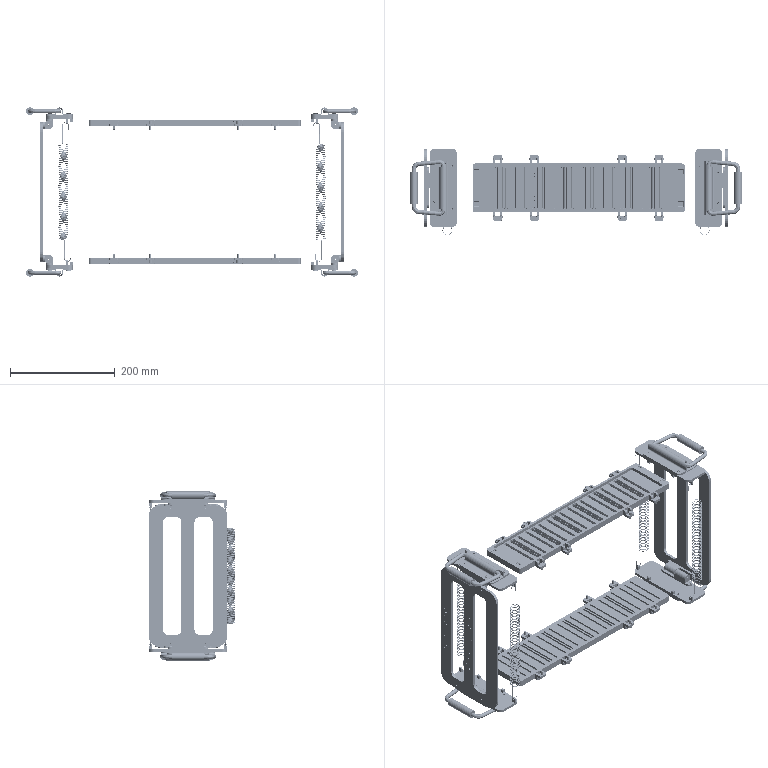Assembly | SolidWorks | mm | 128 component files | 156 solids | 4924 faces | box 634 x 165.5 x 323 mm | volume 1114306 mm3 | plane 2454 | cylinder 1068 | spline 750 | cone 404 | torus 248 | commonest cylinder face diameters 3 x192 3.5 x128 3.4 x96 5.5 x96 5 x72 8 x48 6 x40 2 x40
Bill of materials:
MGL-PACK-01-01WeldPlate1 | 1 |  | Long, thin rectangular plate with rounded corners. The top face has a shallow recessed pocket with many parallel through-slots across the plate's width, plus small square features near the four corners.
MGL-PACK-01-02LocatingBlock | 8 |  | Block with a U-shaped (clevis-like) profile: two upright lugs on a base, each lug with a cross hole. A cylindrical pin with a rounded or chamfered tip sticks out from the underside, and one end of the base is rounded.
MGL-PACK-01-03FixingBlock | 8 |  | U-shaped block similar to the pin-carrying variant: two upright lugs with aligned cross holes, a rounded base end, and a vertical through-hole in the base instead of a protruding pin.
SocketHeadCapScrew_M3_12[GB_T70.1-2000] | 32 |  | Socket-head cap-screw-shaped part: a cylindrical head with a hexagonal socket and a long, plain cylindrical shank with a chamfered tip.
SocketHeadCapScrew_M4_12[GB_T70.1-2000] | 8 |  | Socket-head cap-screw-shaped part with a cylindrical head, a hexagonal socket and a short, plain cylindrical shank with a chamfered end.
MGL-PACK-02-01WeldedPlate2 | 1 |  | Long, thin rectangular plate with rounded corners and many parallel slots spread over its full width, with pairs of small holes on the long edge.
MGL-PACK-03-01FixedPlate | 2 |  | Thin flat frame plate with rounded corners, two large, round-cornered rectangular openings separated by a central bar, and four small holes near the corners.
MGL-PACK-03-02MovingPlate | 4 |  | Flat rectangular plate with fully rounded corners and an asymmetric pattern of round holes: four larger holes, two of them with a smaller hole next to each.
MGL-PACK-03-03SpringSeat | 8 |  | Lug or tab block: rectangular body with a semicircular top end and one large round through-hole centered on the arc.
MGL-PACK-03-04LimitBlock | 8 |  | Solid extruded block with a rectangular lower section and a semicircular or arched top. It has no holes.
MGL-PACK-03-05TensionSpring | 4 |  | Helical coil spring with closely spaced coils and an extended hook formed at each end, consistent with an extension spring.
MGL-PACK-03-06Handle | 4 |  | Folding or drop-style handle: a flat mounting plate with four holes and a curled hinge edge, holding a bent rod in a rectangular U-loop with a cylindrical grip sleeve on the far bar.
MGL-PACK-03-07-01HingePart1 | 4 |  | Flat, thin obround (slot-shaped) plate with a small through-hole near each rounded end. A raised block with a rounded edge (knuckle-like boss) sits on one face along part of the plate's length, offset to one long edge. A slender cylinder (pin) sticks out of the boss end and runs parallel to the plate's long axis, past the boss, for about half the plate length. The overall layout looks like a hinge leaf with a pin.
MGL-PACK-03-07-02HingePart2 | 4 |  | Flat obround plate with a small through-hole near each rounded end. Under one face it has a boss with a rounded end, running along about a third of the plate's length, offset toward one end, with a round through-bore parallel to the plate's long axis. The overall layout looks like a hinge leaf with a knuckle.
PhillipsCountersunkScrewM3_6[GB_T819.1-2000] | 16 |  | Flat-topped countersunk (conical) head with a cross-shaped recess. Below the head is a short necked or filleted transition, then a plain cylindrical shank that ends in a chamfer. The shape looks like a short countersunk screw, but no thread is modeled.
PhillipsCountersunkScrewM5_8[GB_T819.1-2000] | 16 |  | Flat-topped countersunk (conical) head with a cross-shaped recess. Below the head is a necked or filleted transition, then a short plain cylindrical shank that ends in a chamfer. Compared with its head diameter, the shank looks shorter than in unnamed part. The shape looks like a short countersunk screw, but no thread is modeled.
Mates:
1. coincident | MGL-PACK-01-00WeldedPlate1Assembly-1/MGL-PACK-01-01WeldPlate1-1 face at (202.5, 46.5, 12) dir (1, 0, 0) | MGL-PACK-02-00WeldedPlate2Assembly-1/MGL-PACK-02-01WeldedPlate2-1 face at (202.5, 46.5, -263.6) dir (1, 0, 0)
2. coincident | MGL-PACK-01-00WeldedPlate1Assembly-1/MGL-PACK-01-01WeldPlate1-1 face at (-202.5, 46.5, 12) dir (0, 1, 0) | MGL-PACK-02-00WeldedPlate2Assembly-1/MGL-PACK-02-01WeldedPlate2-1 face at (202.5, 46.5, -263.6) dir (0, 1, 0)
3. distance | MGL-PACK-02-00WeldedPlate2Assembly-1/MGL-PACK-02-01WeldedPlate2-1 face at (0, 0, -251.6) dir (0, 0, 1) | MGL-PACK-01-00WeldedPlate1Assembly-1/MGL-PACK-01-01WeldPlate1-1 face at (0, 0, 0) dir (0, 0, -1)
4. distance | MGL-PACK-01-00WeldedPlate1Assembly-1/MGL-PACK-01-01WeldPlate1-1 face at (-202.5, 46.5, 12) dir (0, 1, 0) | MGL-PACK-03-00Fixture-1/MGL-PACK-03-02MovingPlate-1 face at (222.5, 75, 13.7) dir (0, 1, 0)
5. distance | MGL-PACK-03-00Fixture-1/MGL-PACK-03-02MovingPlate-2 face at (222.5, 75, -265.3) dir (-1, 0, 0) | MGL-PACK-02-00WeldedPlate2Assembly-1/MGL-PACK-02-01WeldedPlate2-1 face at (202.5, 46.5, -263.6) dir (1, 0, 0)
6. distance | MGL-PACK-03-00Fixture-2/MGL-PACK-03-02MovingPlate-2 face at (-232.5, 75, 13.7) dir (1, 0, 0) | MGL-PACK-01-00WeldedPlate1Assembly-1/MGL-PACK-01-01WeldPlate1-1 face at (-202.5, 46.5, 12) dir (-1, 0, 0)
7. distance | MGL-PACK-01-00WeldedPlate1Assembly-1/MGL-PACK-01-01WeldPlate1-1 face at (0, 0, 12) dir (0, 0, 1) | MGL-PACK-03-00Fixture-2/MGL-PACK-03-02MovingPlate-2 face at (-258.5, 0, 13.7) dir (0, 0, -1)
8. distance | MGL-PACK-03-00Fixture-1/MGL-PACK-03-02MovingPlate-2 face at (248.5, 0, -265.3) dir (0, 0, 1) | MGL-PACK-02-00WeldedPlate2Assembly-1/MGL-PACK-02-01WeldedPlate2-1 face at (0, 0, -263.6) dir (0, 0, -1)
9. distance | MGL-PACK-01-00WeldedPlate1Assembly-1/MGL-PACK-01-01WeldPlate1-1 face at (-202.5, 46.5, 12) dir (0, 1, 0) | MGL-PACK-03-00Fixture-2/MGL-PACK-03-01FixedPlate-1 face at (-289.5, 75, 8.7) dir (0, 1, 0)
10. coincident | MGL-PACK-01-01WeldPlate1-1 face at (-202.5, 46.5, 12) dir (0, 1, 0) | MGL-PACK-01-02LocatingBlock-1 face at (-163.05, 46.5, 12) dir (0, -1, 0)
11. concentric | MGL-PACK-01-01WeldPlate1-1 face at (-161.05, 46.5, 8.5) dir (0, 1, 0) r 1.5 | MGL-PACK-01-02LocatingBlock-1 face at (-161.05, 53.5, 8.5) dir (0, 1, 0) r 1.7
12. concentric | MGL-PACK-01-01WeldPlate1-1 face at (-148.05, 46.5, 8.5) dir (0, 1, 0) r 1.5 | MGL-PACK-01-02LocatingBlock-1 face at (-148.05, 53.5, 8.5) dir (0, 1, 0) r 1.7
13. coincident | MGL-PACK-01-01WeldPlate1-1 face at (-202.5, 46.5, 12) dir (0, 1, 0) | MGL-PACK-01-02LocatingBlock-9 face at (157.95, 46.5, 12) dir (0, -1, 0)
14. concentric | MGL-PACK-01-01WeldPlate1-1 face at (146.95, 46.5, 8.5) dir (0, 1, 0) r 1.5 | MGL-PACK-01-02LocatingBlock-9 face at (146.95, 53.5, 8.5) dir (0, 1, 0) r 1.7
15. concentric | MGL-PACK-01-01WeldPlate1-1 face at (159.95, 46.5, 8.5) dir (0, 1, 0) r 1.5 | MGL-PACK-01-02LocatingBlock-9 face at (159.95, 53.5, 8.5) dir (0, 1, 0) r 1.7
16. coincident | MGL-PACK-01-01WeldPlate1-1 face at (-202.5, 46.5, 12) dir (0, 1, 0) | MGL-PACK-01-03FixingBlock-1 face at (-93.05, 46.5, 12) dir (0, -1, 0)
17. coincident | MGL-PACK-01-01WeldPlate1-1 face at (-202.5, 46.5, 12) dir (0, 1, 0) | MGL-PACK-01-03FixingBlock-2 face at (87.95, 46.5, 12) dir (0, -1, 0)
18. coincident | MGL-PACK-01-01WeldPlate1-1 face at (-202.5, -46.5, 12) dir (0, -1, 0) | MGL-PACK-01-03FixingBlock-3 face at (-89.05, -46.5, 12) dir (0, 1, 0)
19. coincident | MGL-PACK-01-01WeldPlate1-1 face at (-202.5, -46.5, 12) dir (0, -1, 0) | MGL-PACK-01-03FixingBlock-4 face at (78.95, -46.5, 12) dir (0, 1, 0)
20. concentric | MGL-PACK-01-01WeldPlate1-1 face at (-91.05, 46.5, 8.5) dir (0, 1, 0) r 1.5 | MGL-PACK-01-03FixingBlock-1 face at (-91.05, 53.5, 8.5) dir (0, 1, 0) r 1.7
21. concentric | MGL-PACK-01-01WeldPlate1-1 face at (-78.05, 46.5, 8.5) dir (0, 1, 0) r 1.5 | MGL-PACK-01-03FixingBlock-1 face at (-78.05, 53.5, 8.5) dir (0, 1, 0) r 1.7
22. concentric | MGL-PACK-01-01WeldPlate1-1 face at (89.95, 46.5, 8.5) dir (0, 1, 0) r 1.5 | MGL-PACK-01-03FixingBlock-2 face at (89.95, 53.5, 8.5) dir (0, 1, 0) r 1.7
23. concentric | MGL-PACK-01-01WeldPlate1-1 face at (76.95, 46.5, 8.5) dir (0, 1, 0) r 1.5 | MGL-PACK-01-03FixingBlock-2 face at (76.95, 53.5, 8.5) dir (0, 1, 0) r 1.7
24. coincident | MGL-PACK-01-01WeldPlate1-1 face at (-202.5, -46.5, 12) dir (0, -1, 0) | MGL-PACK-01-02LocatingBlock-13 face at (148.95, -46.5, 12) dir (0, 1, 0)
25. concentric | MGL-PACK-01-01WeldPlate1-1 face at (159.95, 46.5, 8.5) dir (0, 1, 0) r 1.5 | MGL-PACK-01-02LocatingBlock-13 face at (159.95, -53.5, 8.5) dir (0, -1, 0) r 1.7
26. concentric | MGL-PACK-01-01WeldPlate1-1 face at (146.95, 46.5, 8.5) dir (0, 1, 0) r 1.5 | MGL-PACK-01-02LocatingBlock-13 face at (146.95, -53.5, 8.5) dir (0, -1, 0) r 1.7
27. concentric | MGL-PACK-01-01WeldPlate1-1 face at (89.95, 46.5, 8.5) dir (0, 1, 0) r 1.5 | MGL-PACK-01-03FixingBlock-4 face at (89.95, -53.5, 8.5) dir (0, -1, 0) r 1.7
28. concentric | MGL-PACK-01-01WeldPlate1-1 face at (76.95, 46.5, 8.5) dir (0, 1, 0) r 1.5 | MGL-PACK-01-03FixingBlock-4 face at (76.95, -53.5, 8.5) dir (0, -1, 0) r 1.7
29. concentric | MGL-PACK-01-01WeldPlate1-1 face at (-91.05, 46.5, 8.5) dir (0, 1, 0) r 1.5 | MGL-PACK-01-03FixingBlock-3 face at (-91.05, -53.5, 8.5) dir (0, -1, 0) r 1.7
30. concentric | MGL-PACK-01-01WeldPlate1-1 face at (-78.05, 46.5, 8.5) dir (0, 1, 0) r 1.5 | MGL-PACK-01-03FixingBlock-3 face at (-78.05, -53.5, 8.5) dir (0, -1, 0) r 1.7
31. coincident | MGL-PACK-01-01WeldPlate1-1 face at (-202.5, -46.5, 12) dir (0, -1, 0) | MGL-PACK-01-02LocatingBlock-14 face at (-159.05, -46.5, 12) dir (0, 1, 0)
32. concentric | MGL-PACK-01-01WeldPlate1-1 face at (-161.05, 46.5, 8.5) dir (0, 1, 0) r 1.5 | MGL-PACK-01-02LocatingBlock-14 face at (-161.05, -53.5, 8.5) dir (0, -1, 0) r 1.7
33. concentric | MGL-PACK-01-01WeldPlate1-1 face at (-148.05, 46.5, 8.5) dir (0, 1, 0) r 1.5 | MGL-PACK-01-02LocatingBlock-14 face at (-148.05, -53.5, 8.5) dir (0, -1, 0) r 1.7
34. concentric | MGL-PACK-01-03FixingBlock-4 face at (83.45, -58.5, 5) dir (0, 0, 1) r 2.25 | SocketHeadCapScrew_M4_12[GB_T70.1-2000]-1 face at (83.45, -58.5, 9) dir (0, 0, 1) r 2
35. coincident | MGL-PACK-01-03FixingBlock-4 face at (88.95, -59.5, 5) dir (0, 0, 1) | SocketHeadCapScrew_M4_12[GB_T70.1-2000]-1 face at (82.648, -55.093, 5) dir (0, 0, -1)
36. concentric | MGL-PACK-01-03FixingBlock-2 face at (83.45, 58.5, 5) dir (0, 0, 1) r 2.25 | SocketHeadCapScrew_M4_12[GB_T70.1-2000]-4 face at (83.45, 58.5, 9) dir (0, 0, 1) r 2
37. coincident | MGL-PACK-01-03FixingBlock-2 face at (77.95, 59.5, 5) dir (0, 0, 1) | SocketHeadCapScrew_M4_12[GB_T70.1-2000]-4 face at (82.648, 61.907, 5) dir (0, 0, -1)
38. concentric | MGL-PACK-01-02LocatingBlock-13 face at (159.95, -53.5, 8.5) dir (0, -1, 0) r 1.7 | SocketHeadCapScrew_M3_12[GB_T70.1-2000]-1 face at (159.95, -56.5, 8.5) dir (0, -1, 0) r 1.5
39. coincident | MGL-PACK-01-02LocatingBlock-13 face at (144.95, -53.5, 5) dir (0, -1, 0) | SocketHeadCapScrew_M3_12[GB_T70.1-2000]-1 face at (159.407, -53.5, 5.804) dir (0, 1, 0)
40. concentric | MGL-PACK-01-02LocatingBlock-9 face at (159.95, 53.5, 8.5) dir (0, 1, 0) r 1.7 | SocketHeadCapScrew_M3_12[GB_T70.1-2000]-9 face at (159.95, 56.5, 8.5) dir (0, 1, 0) r 1.5
41. coincident | MGL-PACK-01-02LocatingBlock-9 face at (161.95, 53.5, 5) dir (0, 1, 0) | SocketHeadCapScrew_M3_12[GB_T70.1-2000]-9 face at (162.7, 53.5, 8.5) dir (0, -1, 0)
42. concentric | MGL-PACK-01-02LocatingBlock-14 face at (-161.05, -53.5, 8.5) dir (0, -1, 0) r 1.7 | SocketHeadCapScrew_M3_12[GB_T70.1-2000]-13 face at (-161.05, -56.5, 8.5) dir (0, -1, 0) r 1.5
43. coincident | MGL-PACK-01-02LocatingBlock-14 face at (-163.05, -53.5, 5) dir (0, -1, 0) | SocketHeadCapScrew_M3_12[GB_T70.1-2000]-13 face at (-161.926, -53.5, 5.893) dir (0, 1, 0)
44. concentric | MGL-PACK-01-02LocatingBlock-1 face at (-161.05, 53.5, 8.5) dir (0, 1, 0) r 1.7 | SocketHeadCapScrew_M3_12[GB_T70.1-2000]-17 face at (-161.05, 56.5, 8.5) dir (0, 1, 0) r 1.5
45. coincident | MGL-PACK-01-02LocatingBlock-1 face at (-146.05, 53.5, 5) dir (0, 1, 0) | SocketHeadCapScrew_M3_12[GB_T70.1-2000]-17 face at (-160.417, 53.5, 11.176) dir (0, -1, 0)
46. coincident | MGL-PACK-02-01WeldedPlate2-1 face at (-202.5, -46.5, 12) dir (0, -1, 0) | MGL-PACK-01-02LocatingBlock-1 face at (150.05, -46.5, 12) dir (0, 1, 0)
47. concentric | MGL-PACK-02-01WeldedPlate2-1 face at (161.05, -46.5, 8.5) dir (0, -1, 0) r 1.5 | MGL-PACK-01-02LocatingBlock-1 face at (161.05, -53.5, 8.5) dir (0, -1, 0) r 1.7
48. concentric | MGL-PACK-02-01WeldedPlate2-1 face at (148.05, -46.5, 8.5) dir (0, -1, 0) r 1.5 | MGL-PACK-01-02LocatingBlock-1 face at (148.05, -53.5, 8.5) dir (0, -1, 0) r 1.7
49. coincident | MGL-PACK-02-01WeldedPlate2-1 face at (-202.5, -46.5, 12) dir (0, -1, 0) | MGL-PACK-01-02LocatingBlock-9 face at (-144.95, -46.5, 12) dir (0, 1, 0)
50. concentric | MGL-PACK-02-01WeldedPlate2-1 face at (-146.95, -46.5, 8.5) dir (0, -1, 0) r 1.5 | MGL-PACK-01-02LocatingBlock-9 face at (-146.95, -53.5, 8.5) dir (0, -1, 0) r 1.7
51. concentric | MGL-PACK-02-01WeldedPlate2-1 face at (-159.95, -46.5, 8.5) dir (0, -1, 0) r 1.5 | MGL-PACK-01-02LocatingBlock-9 face at (-159.95, -53.5, 8.5) dir (0, -1, 0) r 1.7
52. coincident | MGL-PACK-02-01WeldedPlate2-1 face at (-202.5, -46.5, 12) dir (0, -1, 0) | MGL-PACK-01-03FixingBlock-1 face at (93.05, -46.5, 12) dir (0, 1, 0)
53. coincident | MGL-PACK-02-01WeldedPlate2-1 face at (-202.5, -46.5, 12) dir (0, -1, 0) | MGL-PACK-01-03FixingBlock-2 face at (-87.95, -46.5, 12) dir (0, 1, 0)
54. coincident | MGL-PACK-02-01WeldedPlate2-1 face at (-202.5, 46.5, 12) dir (0, 1, 0) | MGL-PACK-01-03FixingBlock-4 face at (89.05, 46.5, 12) dir (0, -1, 0)
55. coincident | MGL-PACK-02-01WeldedPlate2-1 face at (-202.5, 46.5, 12) dir (0, 1, 0) | MGL-PACK-01-03FixingBlock-5 face at (-78.95, 46.5, 12) dir (0, -1, 0)
56. concentric | MGL-PACK-02-01WeldedPlate2-1 face at (91.05, -46.5, 8.5) dir (0, -1, 0) r 1.5 | MGL-PACK-01-03FixingBlock-1 face at (91.05, -53.5, 8.5) dir (0, -1, 0) r 1.7
57. concentric | MGL-PACK-02-01WeldedPlate2-1 face at (78.05, -46.5, 8.5) dir (0, -1, 0) r 1.5 | MGL-PACK-01-03FixingBlock-1 face at (78.05, -53.5, 8.5) dir (0, -1, 0) r 1.7
58. concentric | MGL-PACK-02-01WeldedPlate2-1 face at (-76.95, -46.5, 8.5) dir (0, -1, 0) r 1.5 | MGL-PACK-01-03FixingBlock-2 face at (-76.95, -53.5, 8.5) dir (0, -1, 0) r 1.7
59. concentric | MGL-PACK-02-01WeldedPlate2-1 face at (-89.95, -46.5, 8.5) dir (0, -1, 0) r 1.5 | MGL-PACK-01-03FixingBlock-2 face at (-89.95, -53.5, 8.5) dir (0, -1, 0) r 1.7
60. coincident | MGL-PACK-02-01WeldedPlate2-1 face at (-202.5, 46.5, 12) dir (0, 1, 0) | MGL-PACK-01-02LocatingBlock-13 face at (-148.95, 46.5, 12) dir (0, -1, 0)
61. concentric | MGL-PACK-02-01WeldedPlate2-1 face at (-159.95, -46.5, 8.5) dir (0, -1, 0) r 1.5 | MGL-PACK-01-02LocatingBlock-13 face at (-159.95, 53.5, 8.5) dir (0, 1, 0) r 1.7
62. concentric | MGL-PACK-02-01WeldedPlate2-1 face at (-146.95, -46.5, 8.5) dir (0, -1, 0) r 1.5 | MGL-PACK-01-02LocatingBlock-13 face at (-146.95, 53.5, 8.5) dir (0, 1, 0) r 1.7
63. concentric | MGL-PACK-02-01WeldedPlate2-1 face at (-89.95, -46.5, 8.5) dir (0, -1, 0) r 1.5 | MGL-PACK-01-03FixingBlock-5 face at (-89.95, 53.5, 8.5) dir (0, 1, 0) r 1.7
64. concentric | MGL-PACK-02-01WeldedPlate2-1 face at (-76.95, -46.5, 8.5) dir (0, -1, 0) r 1.5 | MGL-PACK-01-03FixingBlock-5 face at (-76.95, 53.5, 8.5) dir (0, 1, 0) r 1.7
65. coincident | MGL-PACK-02-01WeldedPlate2-1 face at (-202.5, 46.5, 12) dir (0, 1, 0) | MGL-PACK-01-02LocatingBlock-14 face at (159.05, 46.5, 12) dir (0, -1, 0)
66. concentric | MGL-PACK-02-01WeldedPlate2-1 face at (161.05, -46.5, 8.5) dir (0, -1, 0) r 1.5 | MGL-PACK-01-02LocatingBlock-14 face at (161.05, 53.5, 8.5) dir (0, 1, 0) r 1.7
67. concentric | MGL-PACK-02-01WeldedPlate2-1 face at (148.05, -46.5, 8.5) dir (0, -1, 0) r 1.5 | MGL-PACK-01-02LocatingBlock-14 face at (148.05, 53.5, 8.5) dir (0, 1, 0) r 1.7
68. concentric | MGL-PACK-02-01WeldedPlate2-1 face at (78.05, -46.5, 8.5) dir (0, -1, 0) r 1.5 | MGL-PACK-01-03FixingBlock-4 face at (78.05, 53.5, 8.5) dir (0, 1, 0) r 1.7
69. concentric | MGL-PACK-02-01WeldedPlate2-1 face at (91.05, -46.5, 8.5) dir (0, -1, 0) r 1.5 | MGL-PACK-01-03FixingBlock-4 face at (91.05, 53.5, 8.5) dir (0, 1, 0) r 1.7
70. concentric | MGL-PACK-01-02LocatingBlock-13 face at (-159.95, 53.5, 8.5) dir (0, 1, 0) r 1.7 | SocketHeadCapScrew_M3_12[GB_T70.1-2000]-1 face at (-159.95, 56.5, 8.5) dir (0, 1, 0) r 1.5
71. coincident | MGL-PACK-01-02LocatingBlock-13 face at (-144.95, 53.5, 5) dir (0, 1, 0) | SocketHeadCapScrew_M3_12[GB_T70.1-2000]-1 face at (-159.189, 53.5, 11.143) dir (0, -1, 0)
72. concentric | MGL-PACK-01-02LocatingBlock-9 face at (-159.95, -53.5, 8.5) dir (0, -1, 0) r 1.7 | SocketHeadCapScrew_M3_12[GB_T70.1-2000]-9 face at (-159.95, -56.5, 8.5) dir (0, -1, 0) r 1.5
73. coincident | MGL-PACK-01-02LocatingBlock-9 face at (-161.95, -53.5, 5) dir (0, -1, 0) | SocketHeadCapScrew_M3_12[GB_T70.1-2000]-9 face at (-162.698, -53.5, 8.408) dir (0, 1, 0)
74. concentric | MGL-PACK-01-02LocatingBlock-14 face at (161.05, 53.5, 8.5) dir (0, 1, 0) r 1.7 | SocketHeadCapScrew_M3_12[GB_T70.1-2000]-13 face at (161.05, 56.5, 8.5) dir (0, 1, 0) r 1.5
75. coincident | MGL-PACK-01-02LocatingBlock-14 face at (163.05, 53.5, 5) dir (0, 1, 0) | SocketHeadCapScrew_M3_12[GB_T70.1-2000]-13 face at (163.414, 53.5, 9.905) dir (0, -1, 0)
76. concentric | MGL-PACK-01-02LocatingBlock-1 face at (161.05, -53.5, 8.5) dir (0, -1, 0) r 1.7 | SocketHeadCapScrew_M3_12[GB_T70.1-2000]-17 face at (161.05, -56.5, 8.5) dir (0, -1, 0) r 1.5
77. coincident | MGL-PACK-01-02LocatingBlock-1 face at (146.05, -53.5, 5) dir (0, -1, 0) | SocketHeadCapScrew_M3_12[GB_T70.1-2000]-17 face at (163.233, -53.5, 6.827) dir (0, 1, 0)
78. concentric | MGL-PACK-01-03FixingBlock-5 face at (-83.45, 58.5, 5) dir (0, 0, 1) r 2.25 | SocketHeadCapScrew_M4_12[GB_T70.1-2000]-1 face at (-83.45, 58.5, 9) dir (0, 0, 1) r 2
79. coincident | MGL-PACK-01-03FixingBlock-5 face at (-88.95, 59.5, 5) dir (0, 0, 1) | SocketHeadCapScrew_M4_12[GB_T70.1-2000]-1 face at (-83.477, 62, 5) dir (0, 0, -1)
80. concentric | MGL-PACK-01-03FixingBlock-2 face at (-83.45, -58.5, 5) dir (0, 0, 1) r 2.25 | SocketHeadCapScrew_M4_12[GB_T70.1-2000]-4 face at (-83.45, -58.5, 9) dir (0, 0, 1) r 2
81. coincident | MGL-PACK-01-03FixingBlock-2 face at (-77.95, -59.5, 5) dir (0, 0, 1) | SocketHeadCapScrew_M4_12[GB_T70.1-2000]-4 face at (-82.577, -55.111, 5) dir (0, 0, -1)
82. coincident | MGL-PACK-03-01FixedPlate-1 face at (0, 0, 5) dir (0, 0, 1) | MGL-PACK-03-07Hinge-1/MGL-PACK-03-07-01HingePart1-1 face at (127.5, 32, 5) dir (0, 0, -1)
83. coincident | MGL-PACK-03-01FixedPlate-1 face at (134.5, 75, 5) dir (1, 0, 0) | MGL-PACK-03-07Hinge-1/MGL-PACK-03-07-01HingePart1-1 face at (134.5, 32, 9) dir (1, 0, 0)
84. coincident | MGL-PACK-03-07Hinge-1 plane at (127.5, 0, 5) dir (0, 1, 0) | MGL-PACK-03-00Fixture plane at (0, 0, 0) dir (0, 1, 0)
85. coincident | MGL-PACK-03-01FixedPlate-1 face at (0, 0, 5) dir (0, 0, 1) | MGL-PACK-03-07Hinge-2/MGL-PACK-03-07-01HingePart1-1 face at (-127.5, 32, 5) dir (0, 0, -1)
86. coincident | MGL-PACK-03-01FixedPlate-1 face at (-134.5, 75, 5) dir (-1, 0, 0) | MGL-PACK-03-07Hinge-2/MGL-PACK-03-07-01HingePart1-1 face at (-134.5, 32, 9) dir (-1, 0, 0)
87. coincident | MGL-PACK-03-07Hinge-2/MGL-PACK-03-07-02HingePart2-1 plane at (-139.5, 0, 17) dir (0, -1, 0) | MGL-PACK-03-00Fixture plane at (0, 0, 0) dir (0, 1, 0)
88. coincident | MGL-PACK-03-07Hinge-2/MGL-PACK-03-07-02HingePart2-1 face at (-139.5, -32, 17) dir (-1, 0, 0) | MGL-PACK-03-02MovingPlate-2 face at (-139.5, 0, 36) dir (1, 0, 0)
89. coincident | MGL-PACK-03-07Hinge-2/MGL-PACK-03-07-02HingePart2-1 face at (-135.5, -32, 10) dir (0, 0, -1) | MGL-PACK-03-02MovingPlate-2 face at (-139.5, 75, 10) dir (0, 0, -1)
90. coincident | MGL-PACK-03-07Hinge-2 plane at (-127.5, 0, 5) dir (0, 1, 0) | MGL-PACK-03-02MovingPlate-2 plane at (-144.5, 0, 36) dir (0, 1, 0)
91. coincident | MGL-PACK-03-02MovingPlate-2 face at (-144.5, 0, 36) dir (-1, 0, 0) | MGL-PACK-03-06Handle-2 face at (-144.5, 51.5, 10) dir (1, 0, 0)
92. coincident | MGL-PACK-03-02MovingPlate-2 face at (-139.5, 75, 62) dir (0, 0, 1) | MGL-PACK-03-06Handle-2 face at (-146.5, 42.5, 62) dir (0, 0, 1)
93. coincident | MGL-PACK-03-02MovingPlate-2 plane at (-144.5, 0, 36) dir (0, 1, 0) | MGL-PACK-03-06Handle-2 plane at (-144.5, 0, 36) dir (0, -1, 0)
94. coincident | MGL-PACK-03-02MovingPlate-1 face at (139.5, 0, 36) dir (-1, 0, 0) | MGL-PACK-03-07Hinge-1/MGL-PACK-03-07-02HingePart2-1 face at (139.5, -32, 17) dir (1, 0, 0)
95. coincident | MGL-PACK-03-02MovingPlate-1 face at (139.5, -75, 10) dir (0, 0, -1) | MGL-PACK-03-07Hinge-1/MGL-PACK-03-07-02HingePart2-1 face at (135.5, -32, 10) dir (0, 0, -1)
96. coincident | MGL-PACK-03-02MovingPlate-1 face at (144.5, 0, 36) dir (1, 0, 0) | MGL-PACK-03-06Handle-1 face at (144.5, -51.5, 10) dir (-1, 0, 0)
97. coincident | MGL-PACK-03-02MovingPlate-1 face at (139.5, -75, 62) dir (0, 0, 1) | MGL-PACK-03-06Handle-1 face at (146.5, -42.5, 62) dir (0, 0, 1)
98. coincident | MGL-PACK-03-02MovingPlate-1 plane at (144.5, 0, 36) dir (0, -1, 0) | MGL-PACK-03-07Hinge-1 plane at (127.5, 0, 5) dir (0, 1, 0)
99. coincident | MGL-PACK-03-02MovingPlate-1 plane at (144.5, 0, 36) dir (0, -1, 0) | MGL-PACK-03-06Handle-1 plane at (144.5, 0, 36) dir (0, 1, 0)
100. coincident | MGL-PACK-03-02MovingPlate-2 face at (-139.5, 0, 36) dir (1, 0, 0) | MGL-PACK-03-03SpringSeat-1 face at (-139.5, 75, 52) dir (-1, 0, 0)
101. coincident | MGL-PACK-03-02MovingPlate-2 face at (-139.5, 75, 62) dir (0, 1, 0) | MGL-PACK-03-03SpringSeat-1 face at (-139.5, 75, 52) dir (0, 1, 0)
102. distance | MGL-PACK-03-03SpringSeat-1 face at (-132.5, 72, 52) dir (0, 0, 1) | MGL-PACK-03-02MovingPlate-2 face at (-139.5, 75, 62) dir (0, 0, 1)
103. coincident | MGL-PACK-03-02MovingPlate-1 face at (139.5, 0, 36) dir (-1, 0, 0) | MGL-PACK-03-03SpringSeat-4 face at (139.5, 75, 49) dir (1, 0, 0)
104. coincident | MGL-PACK-03-02MovingPlate-1 face at (139.5, 75, 62) dir (0, 1, 0) | MGL-PACK-03-03SpringSeat-4 face at (139.5, 75, 49) dir (0, 1, 0)
105. distance | MGL-PACK-03-03SpringSeat-4 face at (132.5, 72, 52) dir (0, 0, 1) | MGL-PACK-03-02MovingPlate-1 face at (139.5, -75, 62) dir (0, 0, 1)
106. distance | MGL-PACK-03-05TensionSpring-1 plane at (-91.5, 63, 44) dir (-1, 0, 0) | MGL-PACK-03-02MovingPlate-2 face at (-139.5, 0, 36) dir (1, 0, 0)
107. distance | MGL-PACK-03-05TensionSpring-1 plane at (-91.5, 63, 44) dir (0, 1, 0) | MGL-PACK-03-02MovingPlate-2 face at (-139.5, 75, 62) dir (0, 1, 0)
108. distance | MGL-PACK-03-05TensionSpring-1 plane at (-91.5, 63, 44) dir (0, 0, 1) | MGL-PACK-03-03SpringSeat-4 face at (132.5, 72, 49) dir (0, 0, -1)
109. concentric | MGL-PACK-03-02MovingPlate-1 face at (144.5, 41, 54) dir (1, 0, 0) r 2.5 | PhillipsCountersunkScrewM5_8[GB_T819.1-2000]-1 face at (150.3, 41, 54) dir (1, 0, 0) r 2.5
110. distance | MGL-PACK-03-06Handle-1 edge at (148.5, 42.5, 62) dir (0, -1, 0) | PhillipsCountersunkScrewM5_8[GB_T819.1-2000]-1 face at (150.3, 41, 54) dir (1, 0, 0)
111. concentric | MGL-PACK-03-02MovingPlate-1 face at (144.5, 28.5, 18) dir (1, 0, 0) r 2.5 | PhillipsCountersunkScrewM5_8[GB_T819.1-2000]-7 face at (150.4, 28.5, 18) dir (1, 0, 0) r 2.5
112. concentric | MGL-PACK-03-02MovingPlate-2 face at (-144.5, 41, 54) dir (-1, 0, 0) r 2.5 | PhillipsCountersunkScrewM5_8[GB_T819.1-2000]-9 face at (-150.4, 41, 54) dir (-1, 0, 0) r 2.5
113. distance | MGL-PACK-03-06Handle-2 face at (-148.5, 51.5, 62) dir (-1, 0, 0) | PhillipsCountersunkScrewM5_8[GB_T819.1-2000]-9 face at (-150.4, 41, 54) dir (-1, 0, 0)
114. distance | PhillipsCountersunkScrewM5_8[GB_T819.1-2000]-7 face at (150.4, 28.5, 18) dir (1, 0, 0) | MGL-PACK-03-06Handle-1 face at (148.5, -40, 26.5) dir (1, 0, 0)
115. concentric | MGL-PACK-03-02MovingPlate-2 face at (-144.5, 28.5, 18) dir (-1, 0, 0) r 2.5 | PhillipsCountersunkScrewM5_8[GB_T819.1-2000]-11 face at (-150.4, 28.5, 18) dir (-1, 0, 0) r 2.5
116. coincident | PhillipsCountersunkScrewM5_8[GB_T819.1-2000]-9 face at (-150.4, 41, 54) dir (-1, 0, 0) | PhillipsCountersunkScrewM5_8[GB_T819.1-2000]-11 face at (-150.4, 28.5, 18) dir (-1, 0, 0)
117. concentric | MGL-PACK-03-07Hinge-2/MGL-PACK-03-07-02HingePart2-1 face at (-135.5, 33.5, 17) dir (1, 0, 0) r 1.7 | PhillipsCountersunkScrewM3_6[GB_T819.1-2000]-1 face at (-135.5, 33.5, 17) dir (1, 0, 0) r 1.5
118. coincident | MGL-PACK-03-07Hinge-2/MGL-PACK-03-07-02HingePart2-1 face at (-135.5, -32, 17) dir (1, 0, 0) | PhillipsCountersunkScrewM3_6[GB_T819.1-2000]-1 face at (-135.5, 33.5, 17) dir (1, 0, 0)
119. concentric | MGL-PACK-03-07Hinge-2/MGL-PACK-03-07-01HingePart1-1 face at (-127.5, 33.5, 9) dir (0, 0, 1) r 1.7 | PhillipsCountersunkScrewM3_6[GB_T819.1-2000]-6 face at (-127.5, 33.5, 9) dir (0, 0, 1) r 1.5
120. coincident | MGL-PACK-03-07Hinge-2/MGL-PACK-03-07-01HingePart1-1 face at (-127.5, 32, 9) dir (0, 0, 1) | PhillipsCountersunkScrewM3_6[GB_T819.1-2000]-6 face at (-127.5, 33.5, 9) dir (0, 0, 1)
121. concentric | MGL-PACK-03-07Hinge-1/MGL-PACK-03-07-02HingePart2-1 face at (135.5, 33.5, 17) dir (-1, 0, 0) r 1.7 | PhillipsCountersunkScrewM3_6[GB_T819.1-2000]-8 face at (135.5, 33.5, 17) dir (-1, 0, 0) r 1.5
122. coincident | MGL-PACK-03-07Hinge-1/MGL-PACK-03-07-02HingePart2-1 face at (135.5, -32, 17) dir (-1, 0, 0) | PhillipsCountersunkScrewM3_6[GB_T819.1-2000]-8 face at (135.5, 33.5, 17) dir (-1, 0, 0)
123. concentric | MGL-PACK-03-07Hinge-1/MGL-PACK-03-07-01HingePart1-1 face at (127.5, 33.5, 9) dir (0, 0, 1) r 1.7 | PhillipsCountersunkScrewM3_6[GB_T819.1-2000]-10 face at (127.5, 33.5, 9) dir (0, 0, 1) r 1.5
124. coincident | MGL-PACK-03-07Hinge-1/MGL-PACK-03-07-01HingePart1-1 face at (127.5, 32, 9) dir (0, 0, 1) | PhillipsCountersunkScrewM3_6[GB_T819.1-2000]-10 face at (127.5, 33.5, 9) dir (0, 0, 1)
125. perpendicular | MGL-PACK-03-01FixedPlate-1 face at (0, 0, 0) dir (0, 0, -1) | MGL-PACK-03-02MovingPlate-2 face at (-144.5, 0, 36) dir (-1, 0, 0)
126. parallel | MGL-PACK-03-02MovingPlate-1 face at (144.5, 0, 36) dir (1, 0, 0) | MGL-PACK-03-02MovingPlate-2 face at (-144.5, 0, 36) dir (-1, 0, 0)
127. coincident | MGL-PACK-03-02MovingPlate-2 face at (-139.5, 0, 36) dir (1, 0, 0) | MGL-PACK-03-04LimitBlock-1 face at (-139.5, 35, 57) dir (-1, 0, 0)
128. coincident | MGL-PACK-03-02MovingPlate-2 face at (-139.5, 75, 62) dir (0, 0, 1) | MGL-PACK-03-04LimitBlock-1 face at (-139.5, 35, 62) dir (0, 0, 1)
129. distance | MGL-PACK-03-04LimitBlock-1 face at (-135.5, 35, 59.5) dir (0, 1, 0) | MGL-PACK-03-02MovingPlate-2 face at (-139.5, 75, 62) dir (0, 1, 0)
130. coincident | MGL-PACK-03-02MovingPlate-1 face at (139.5, 0, 36) dir (-1, 0, 0) | MGL-PACK-03-04LimitBlock-3 face at (139.5, 30, 57) dir (1, 0, 0)
131. coincident | MGL-PACK-03-02MovingPlate-1 face at (139.5, -75, 62) dir (0, 0, 1) | MGL-PACK-03-04LimitBlock-3 face at (139.5, 30, 62) dir (0, 0, 1)
132. distance | MGL-PACK-03-02MovingPlate-1 face at (139.5, 75, 62) dir (0, 1, 0) | MGL-PACK-03-04LimitBlock-3 face at (135.5, 35, 59.5) dir (0, 1, 0)
133. concentric | MGL-PACK-03-07-01HingePart1-1 face at (0, -28.5, 12) dir (0, 1, 0) r 2 | MGL-PACK-03-07-02HingePart2-1 face at (0, -0.5, 12) dir (0, -1, 0) r 2.1
134. distance | MGL-PACK-03-07-01HingePart1-1 face at (0, 0.5, 12) dir (0, -1, 0) | MGL-PACK-03-07-02HingePart2-1 face at (0, -0.5, 12) dir (0, 1, 0)